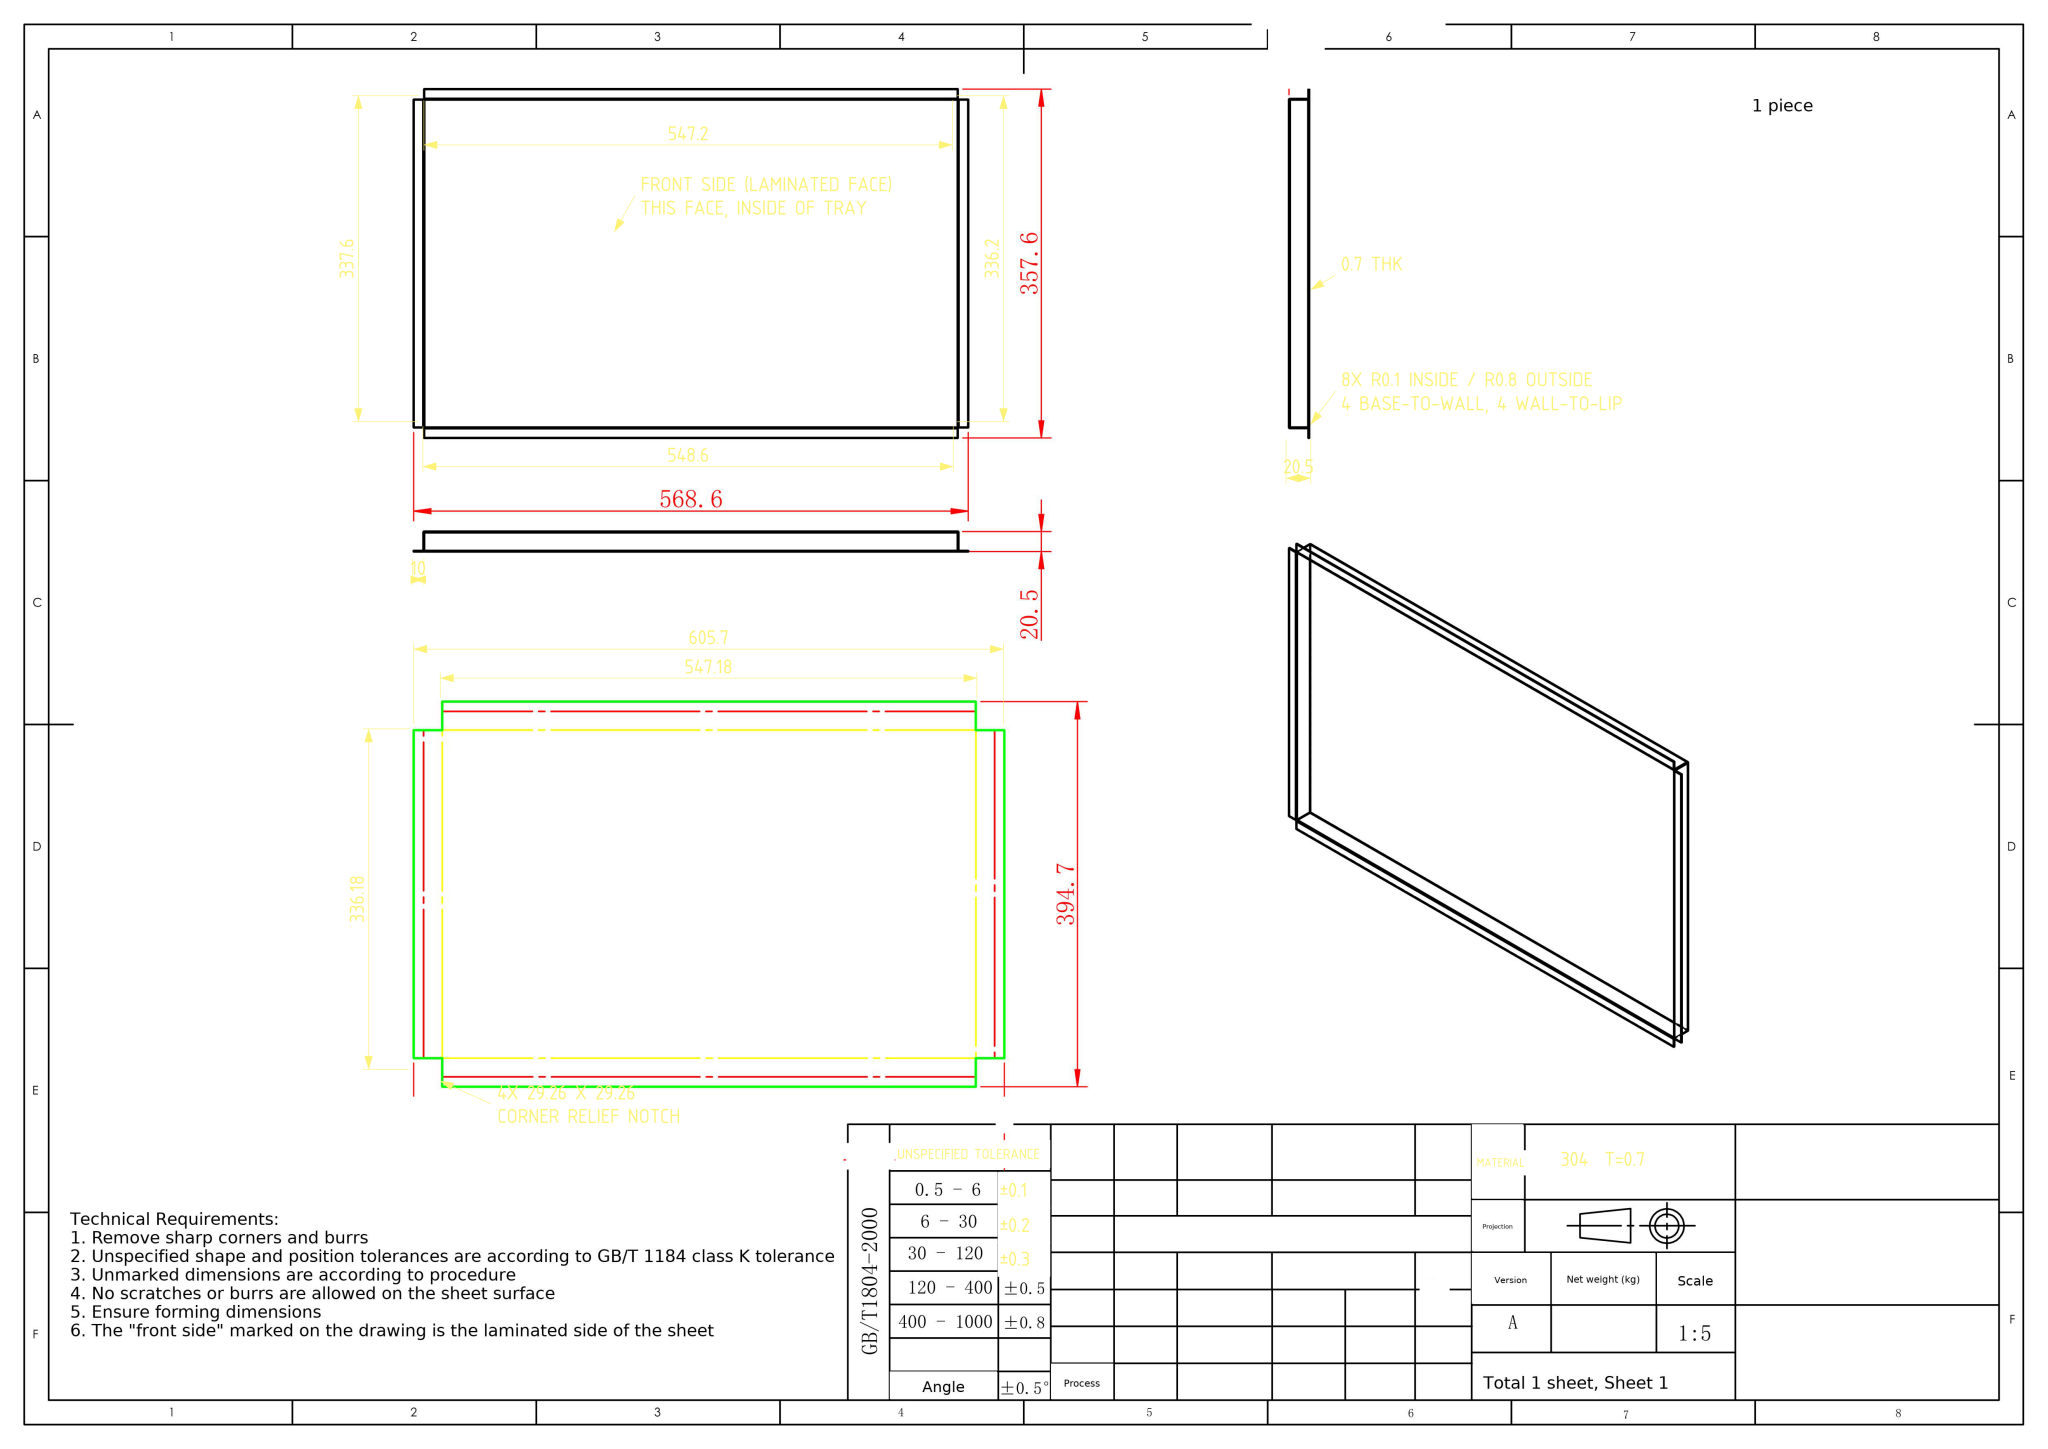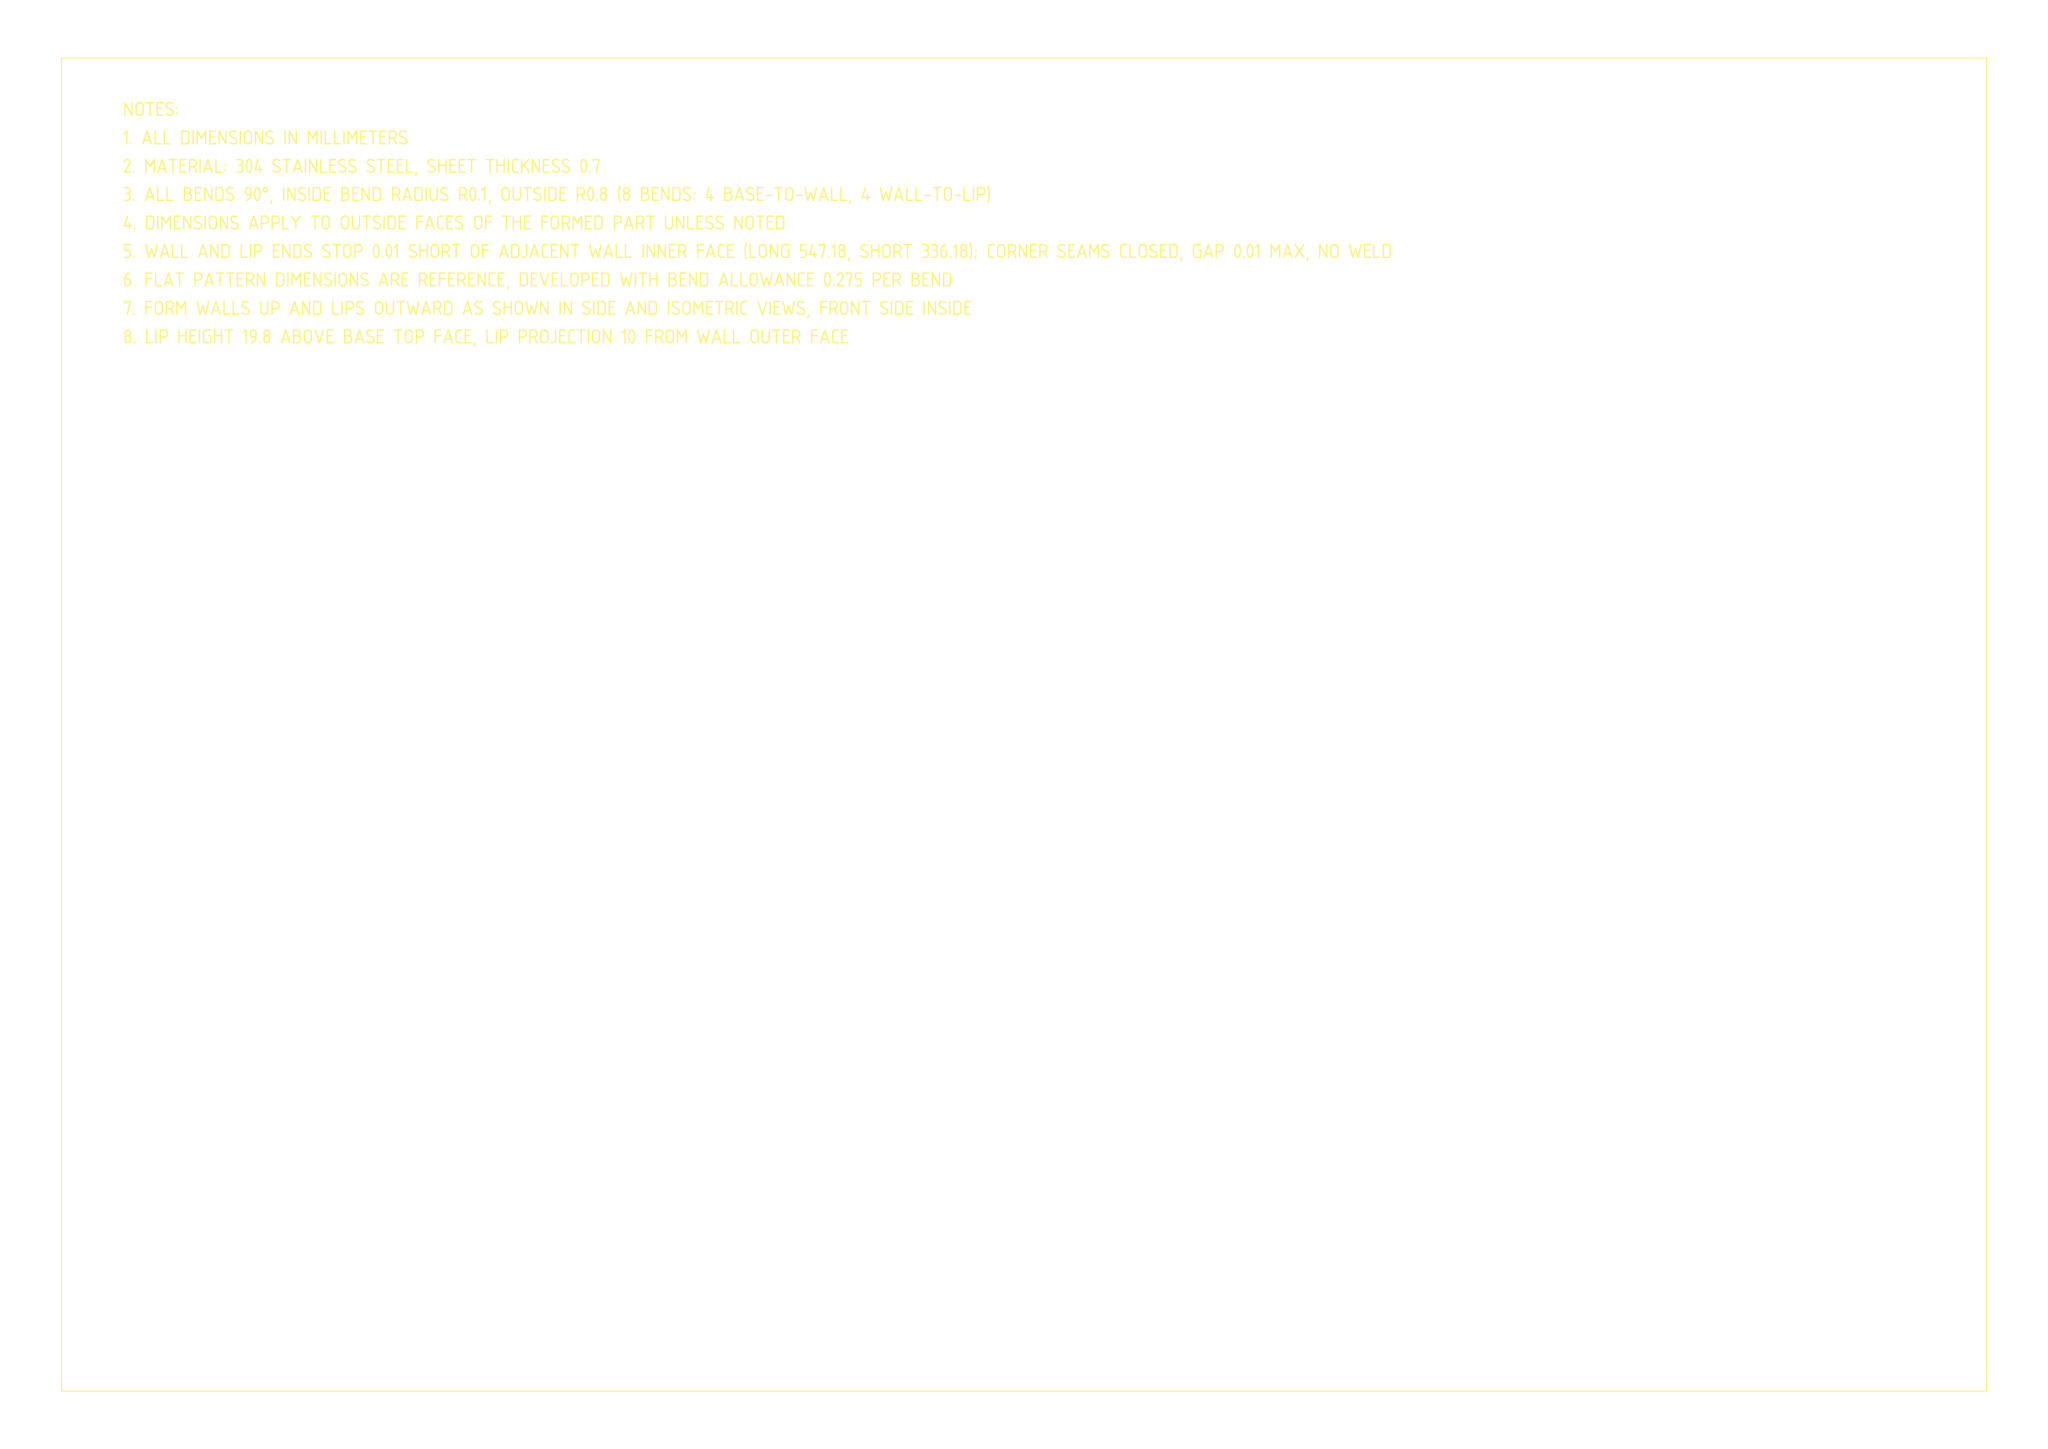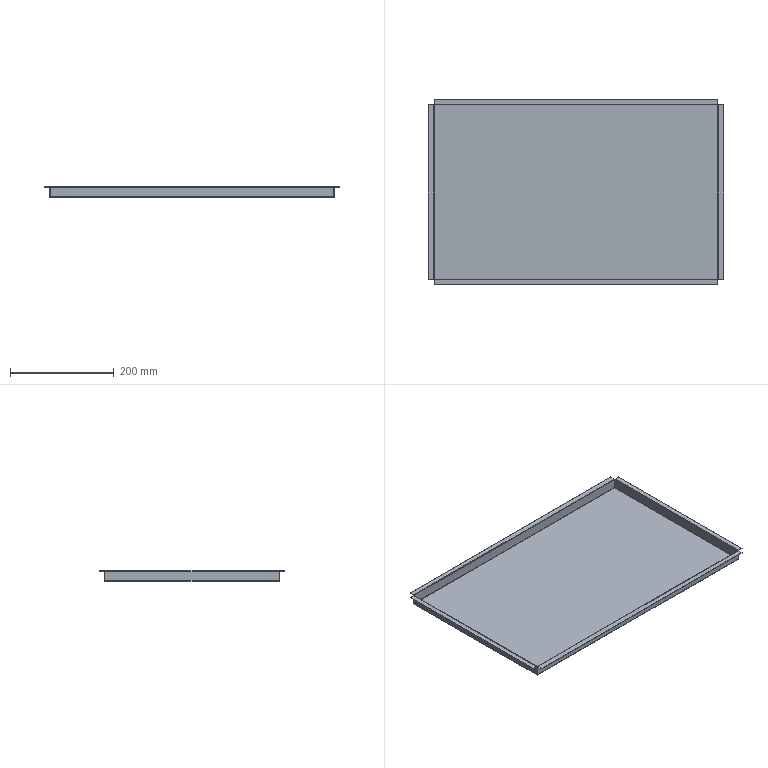Part | NX | mm | 1 solid | 70 faces | box 568.6 x 357.6 x 20.5 mm | volume 166020 mm3 | plane 46 | cylinder 16 | spline 8 | commonest cylinder face diameters 1.6 x8 0.2 x8